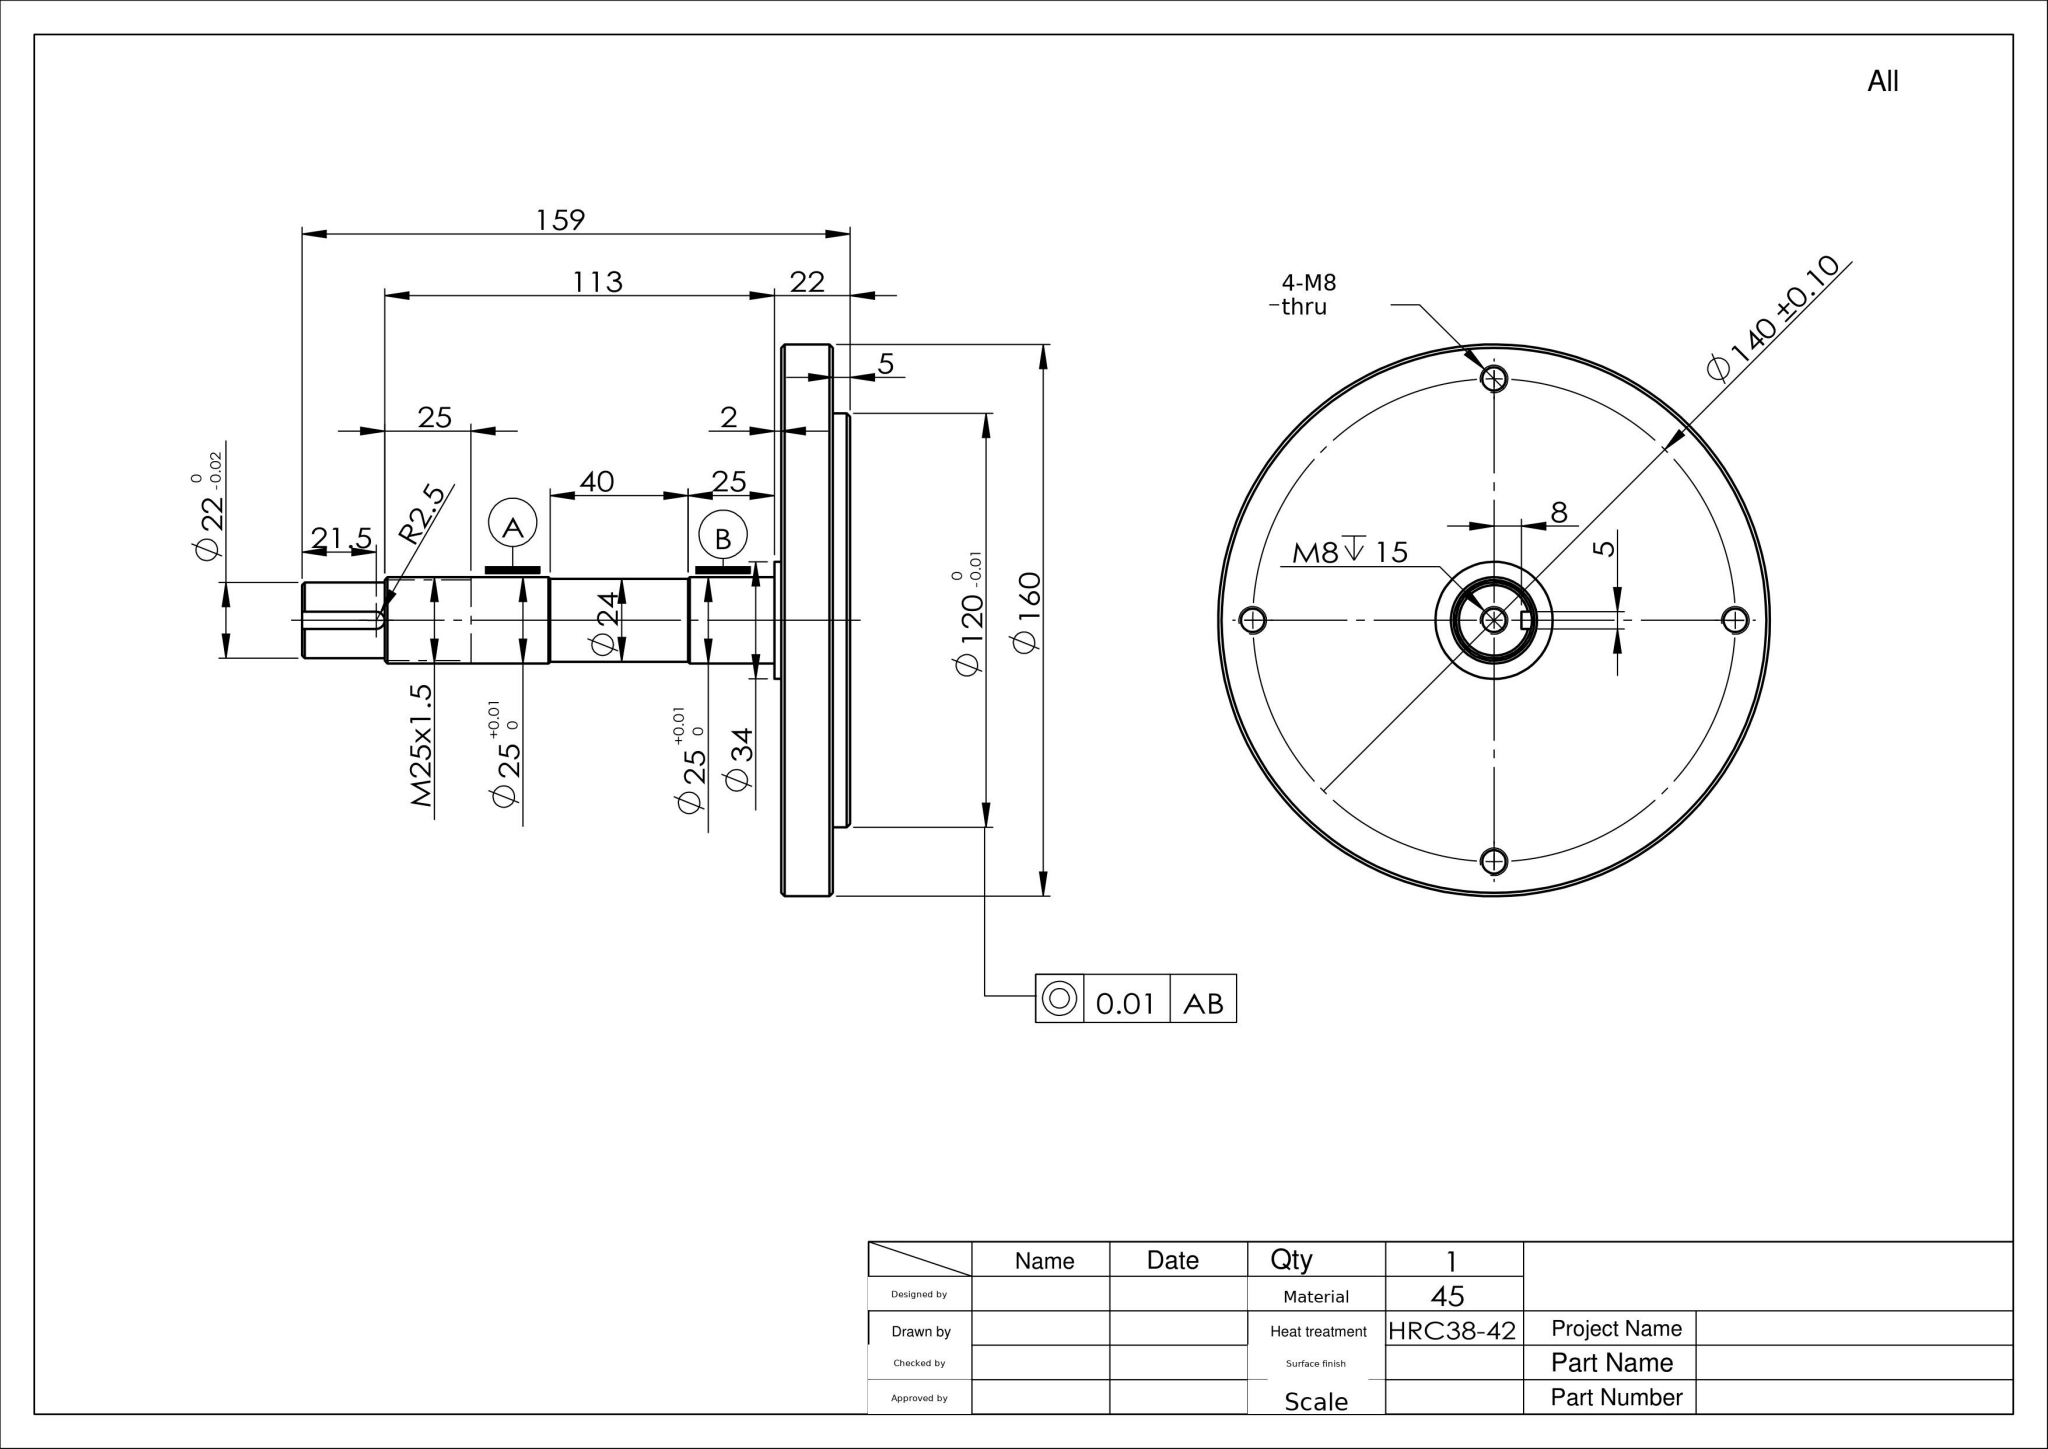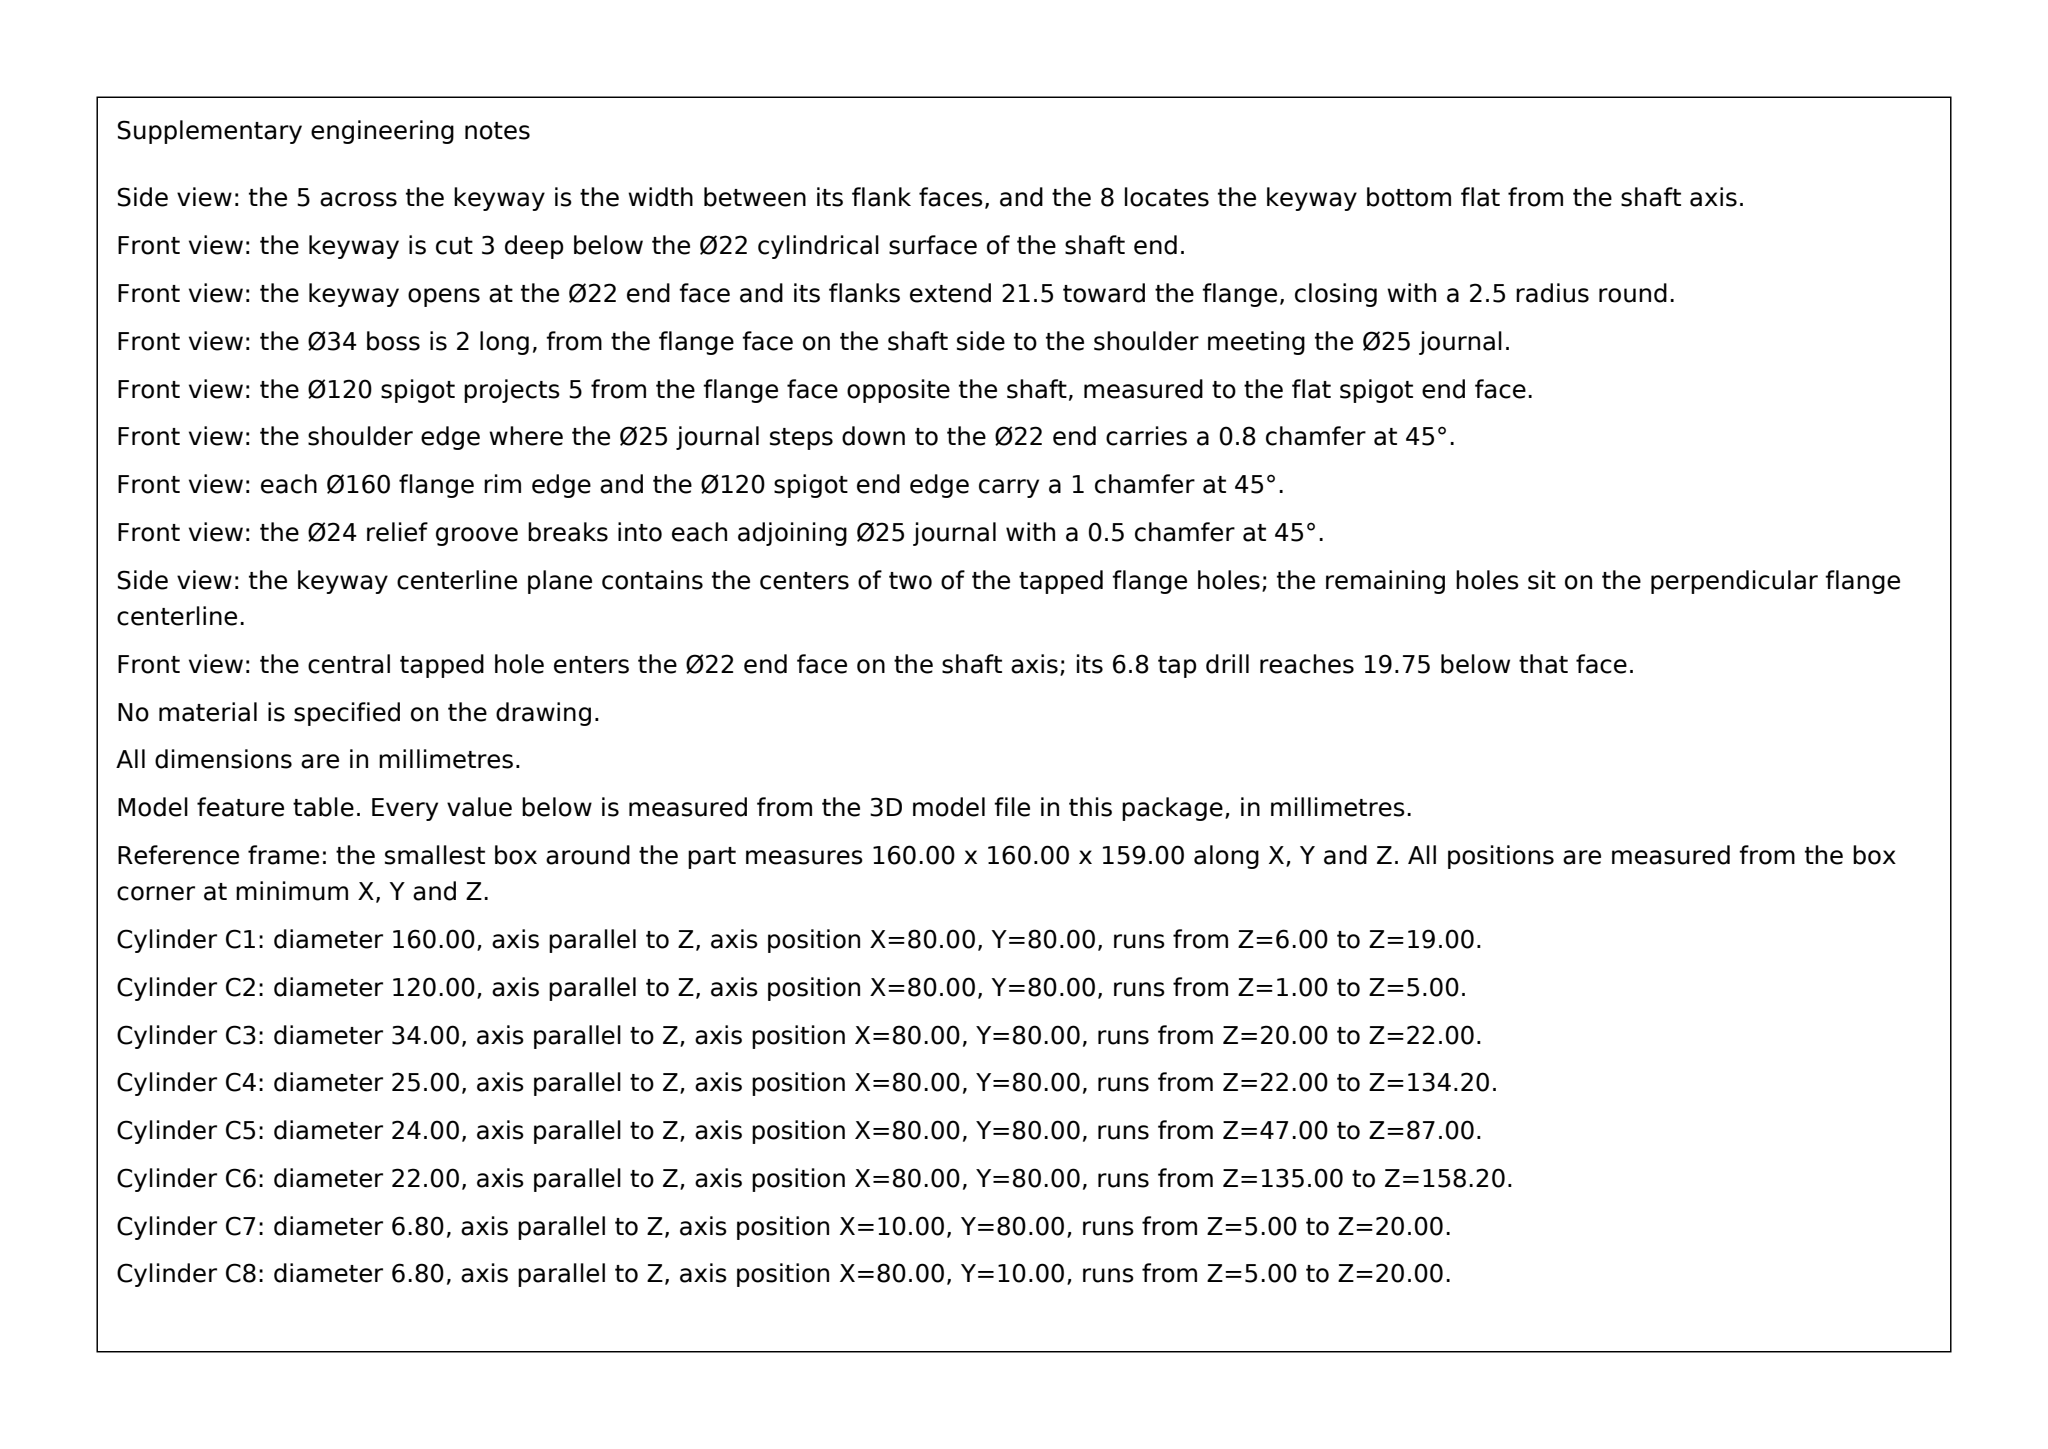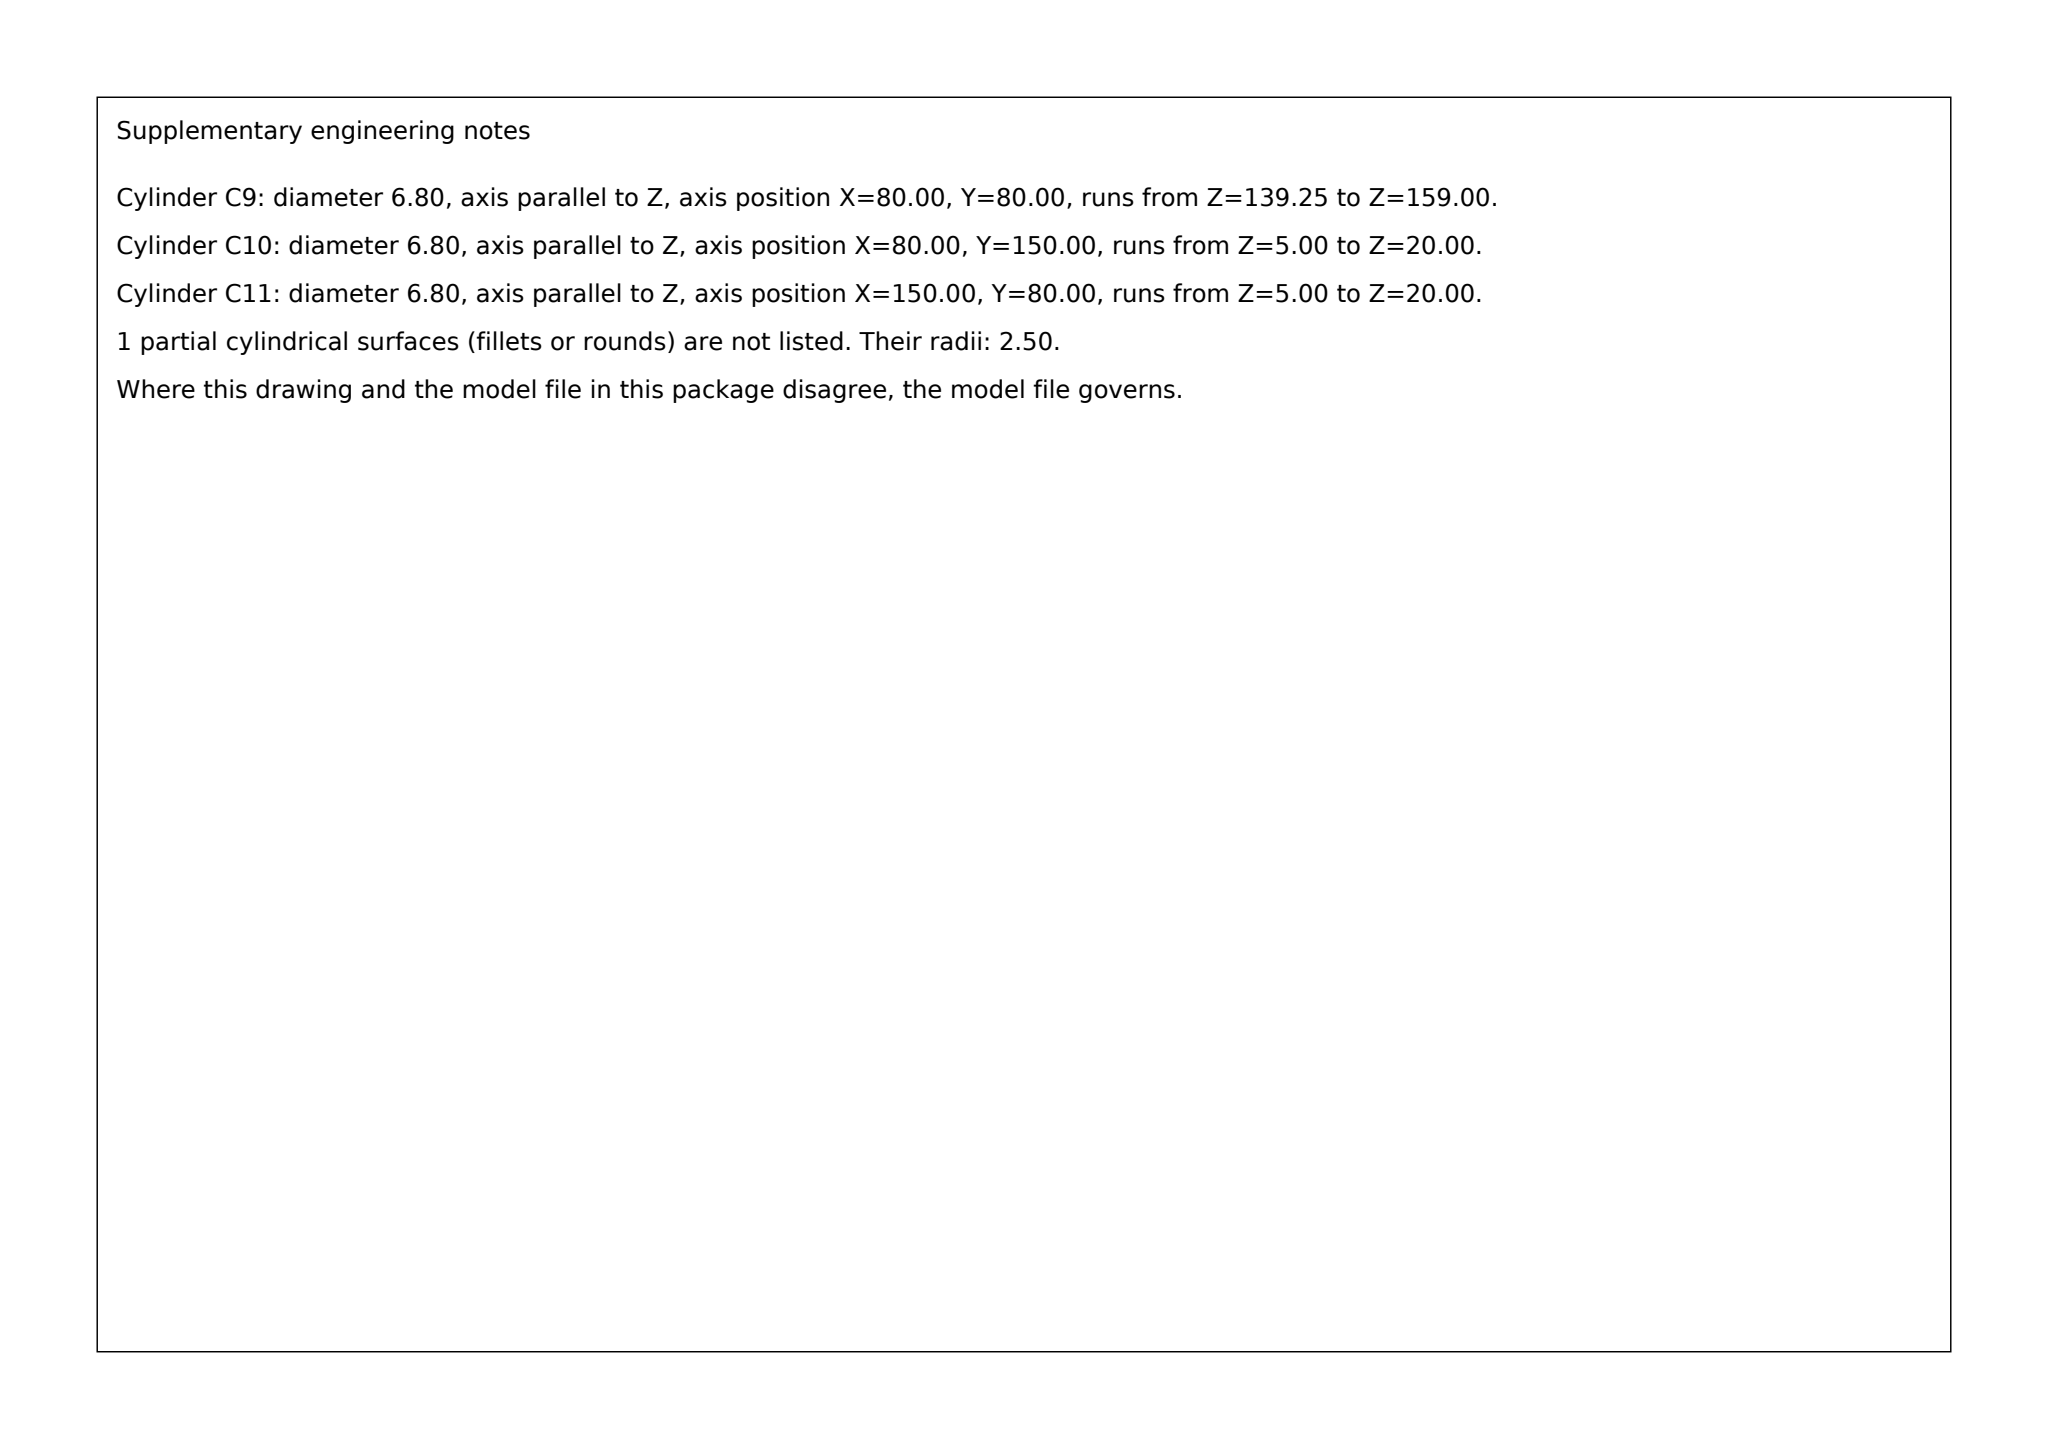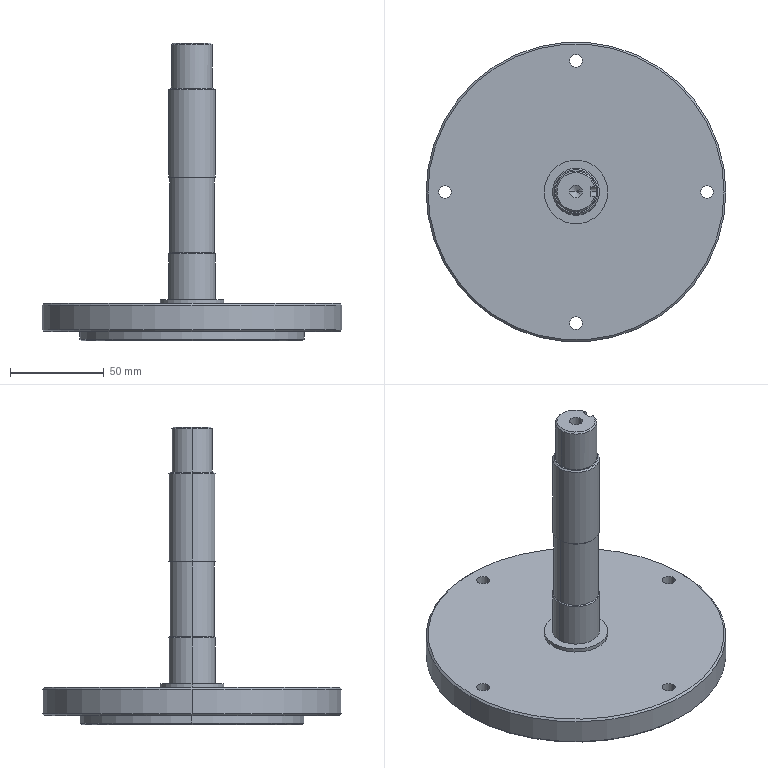Part | SolidWorks | mm | material 45 | 1 solid | 51 faces | box 160 x 160 x 159 mm | volume 418996 mm3 | cylinder 26 | cone 16 | plane 9 | commonest cylinder face diameters 6.8 x10 25 x4 22 x2 5 x2 24 x2 120 x2 34 x2 160 x2
Drawing notes:
Ø22 SHAFT END CHAMFER C0.8 | from the solid: Cone 90 deg, ref dia 20.4, at z=158.2, size 0.8 (Ø22 free end)
Ø25 TO Ø22 STEP CHAMFER C0.8 | from the solid: Cone 90 deg, ref dia 23.4, at z=134.2, size 0.8 (end of Ø25 journal)
Ø25/Ø24 STEP CHAMFERS C0.5, 2 PLCS | from the solid: Cones 90 deg, ref dia 25.0 at z=46.5 and z=87.0, size 0.5
Ø160 FLANGE OD EDGES C1, BOTH ENDS | from the solid: Cones 90 deg ref dia 160 at z=5 and ref dia 158 at z=19, size 1.0
Ø120 SPIGOT EDGE C1 | from the solid: Cone 90 deg, ref dia 118, at z=0, size 1.0 (Ø120 boss z=1-5)
4X M8 THRU ON Ø140 B.C. (Ø6.8 DRILL THRU 15 THK) | from the solid: 4 holes Ø6.8 at x/y 10 & 150 (R70 = Ø140 B.C.), z=5 to 20, thru flange
CENTER: M8 DP 15, Ø6.8 DRILL DP 19.7 IN Ø22 SHAFT END | from the solid: Ø6.8 bore on axis (80,80), z=139.3 to 159.0 = 19.7 deep, 118 deg point